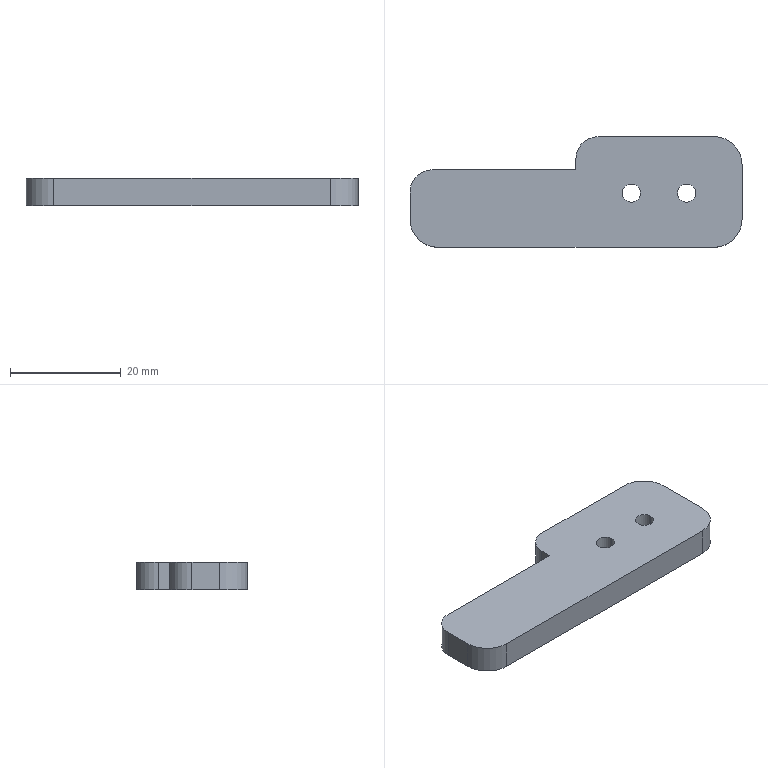Component | SolidWorks | 3UpperBaffle-FrontSmallBaffle9.26-1 | 1 solid | 17 faces | volume 4900 mm3 | cylinder 9 | plane 8 | commonest cylinder face diameters 3.3 x4 10 x3 8 x2 | material AISI 1045 Steel, Cold Drawn